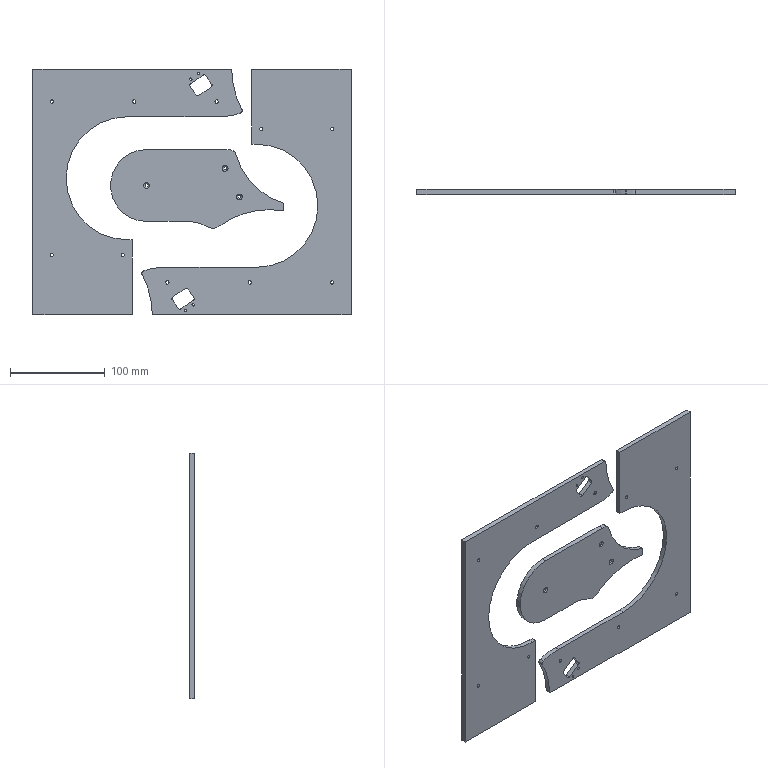CAM job | Mastercam | mm | 4 operations | part box 336 x 5 x 259
1. Contour (Ramp) | 3 - 3 平铣刀
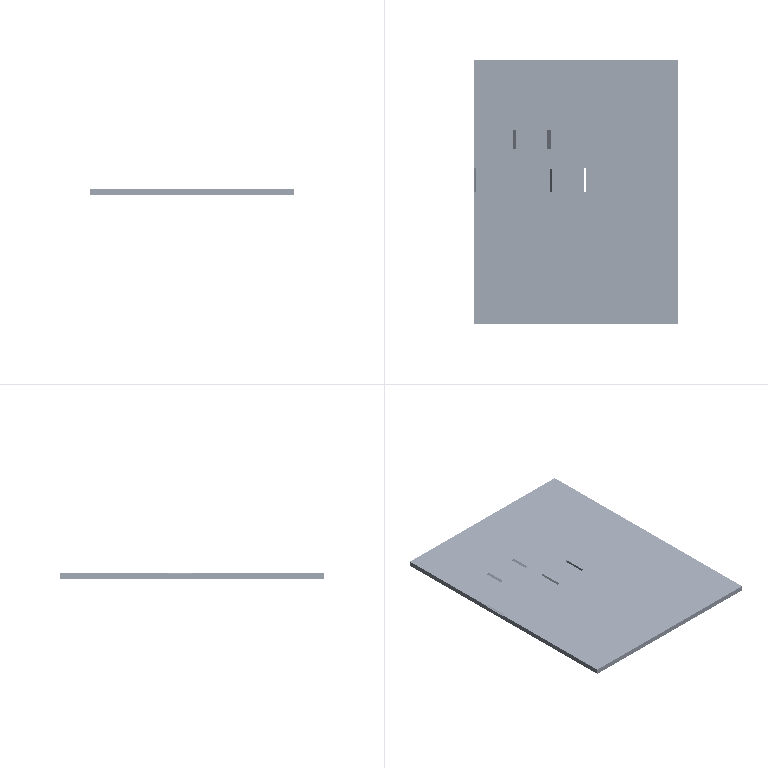2. Contour (2D) | 3 - 3 平铣刀
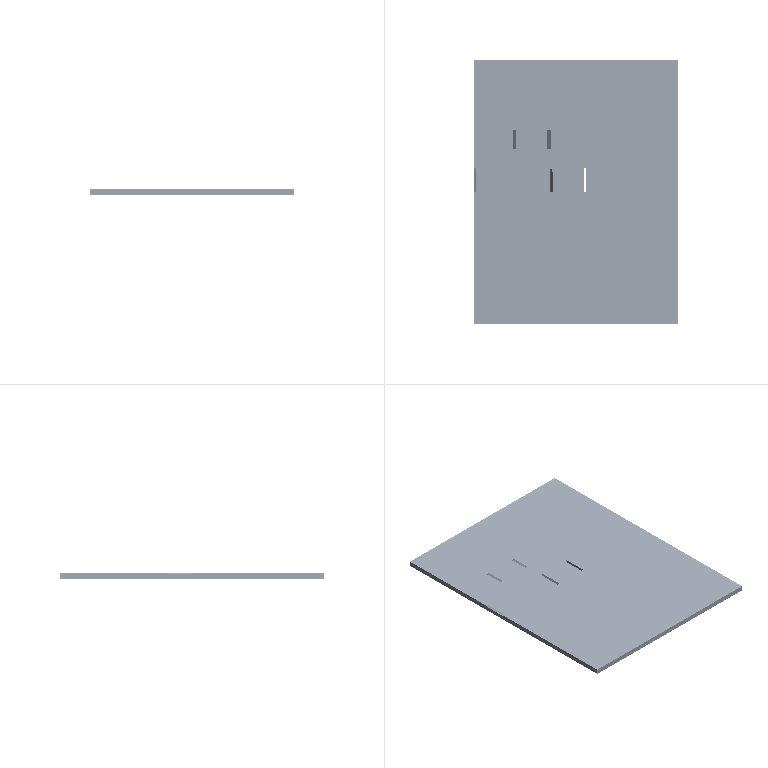3. Drill/Counterbore | 7 - 4 倒角刀
4. Contour (2D chamfer) | 7 - 4 倒角刀